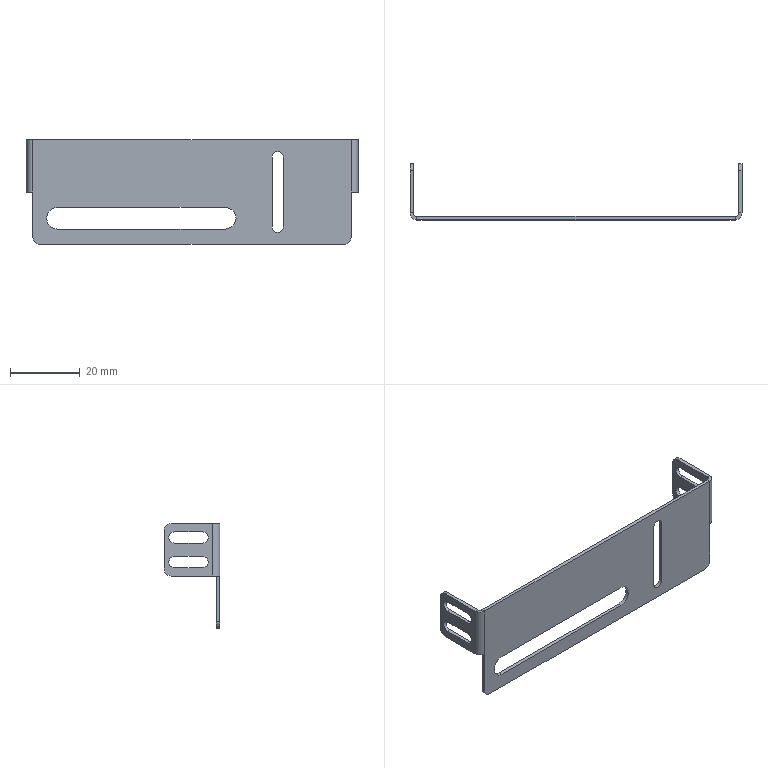Component | SolidWorks | B-TRD899MINI-2213-01FiberOpticBracket-1 | 1 solid | 55 faces | volume 2681 mm3 | plane 32 | cylinder 23 | commonest cylinder face diameters 3.2 x10 4 x8 6.2 x3 2 x2 | material SUS201